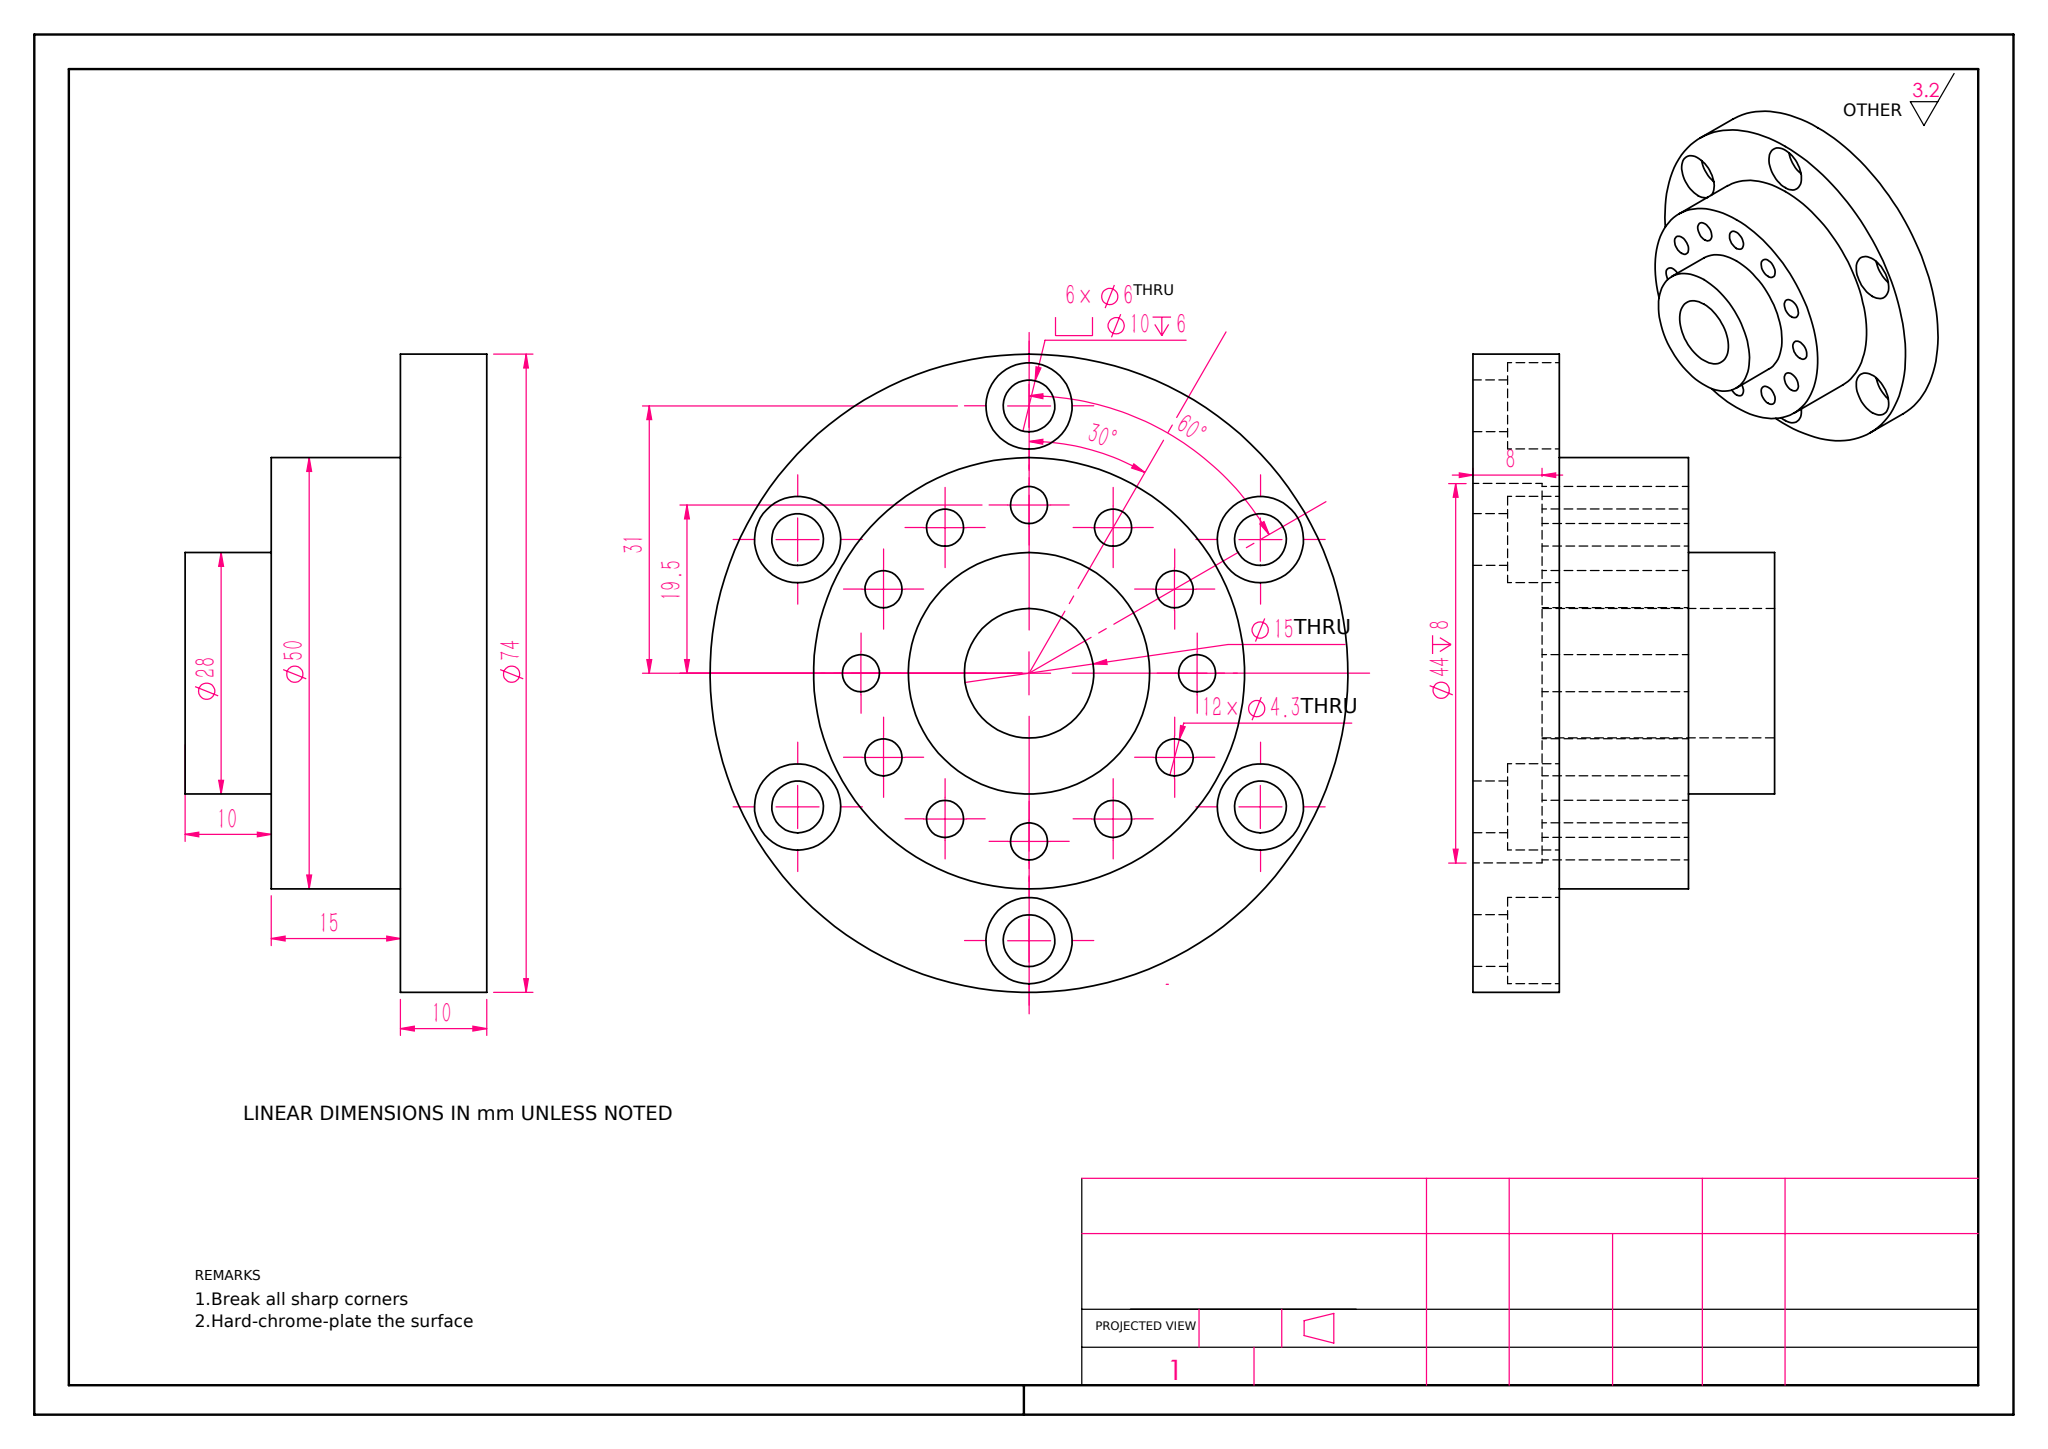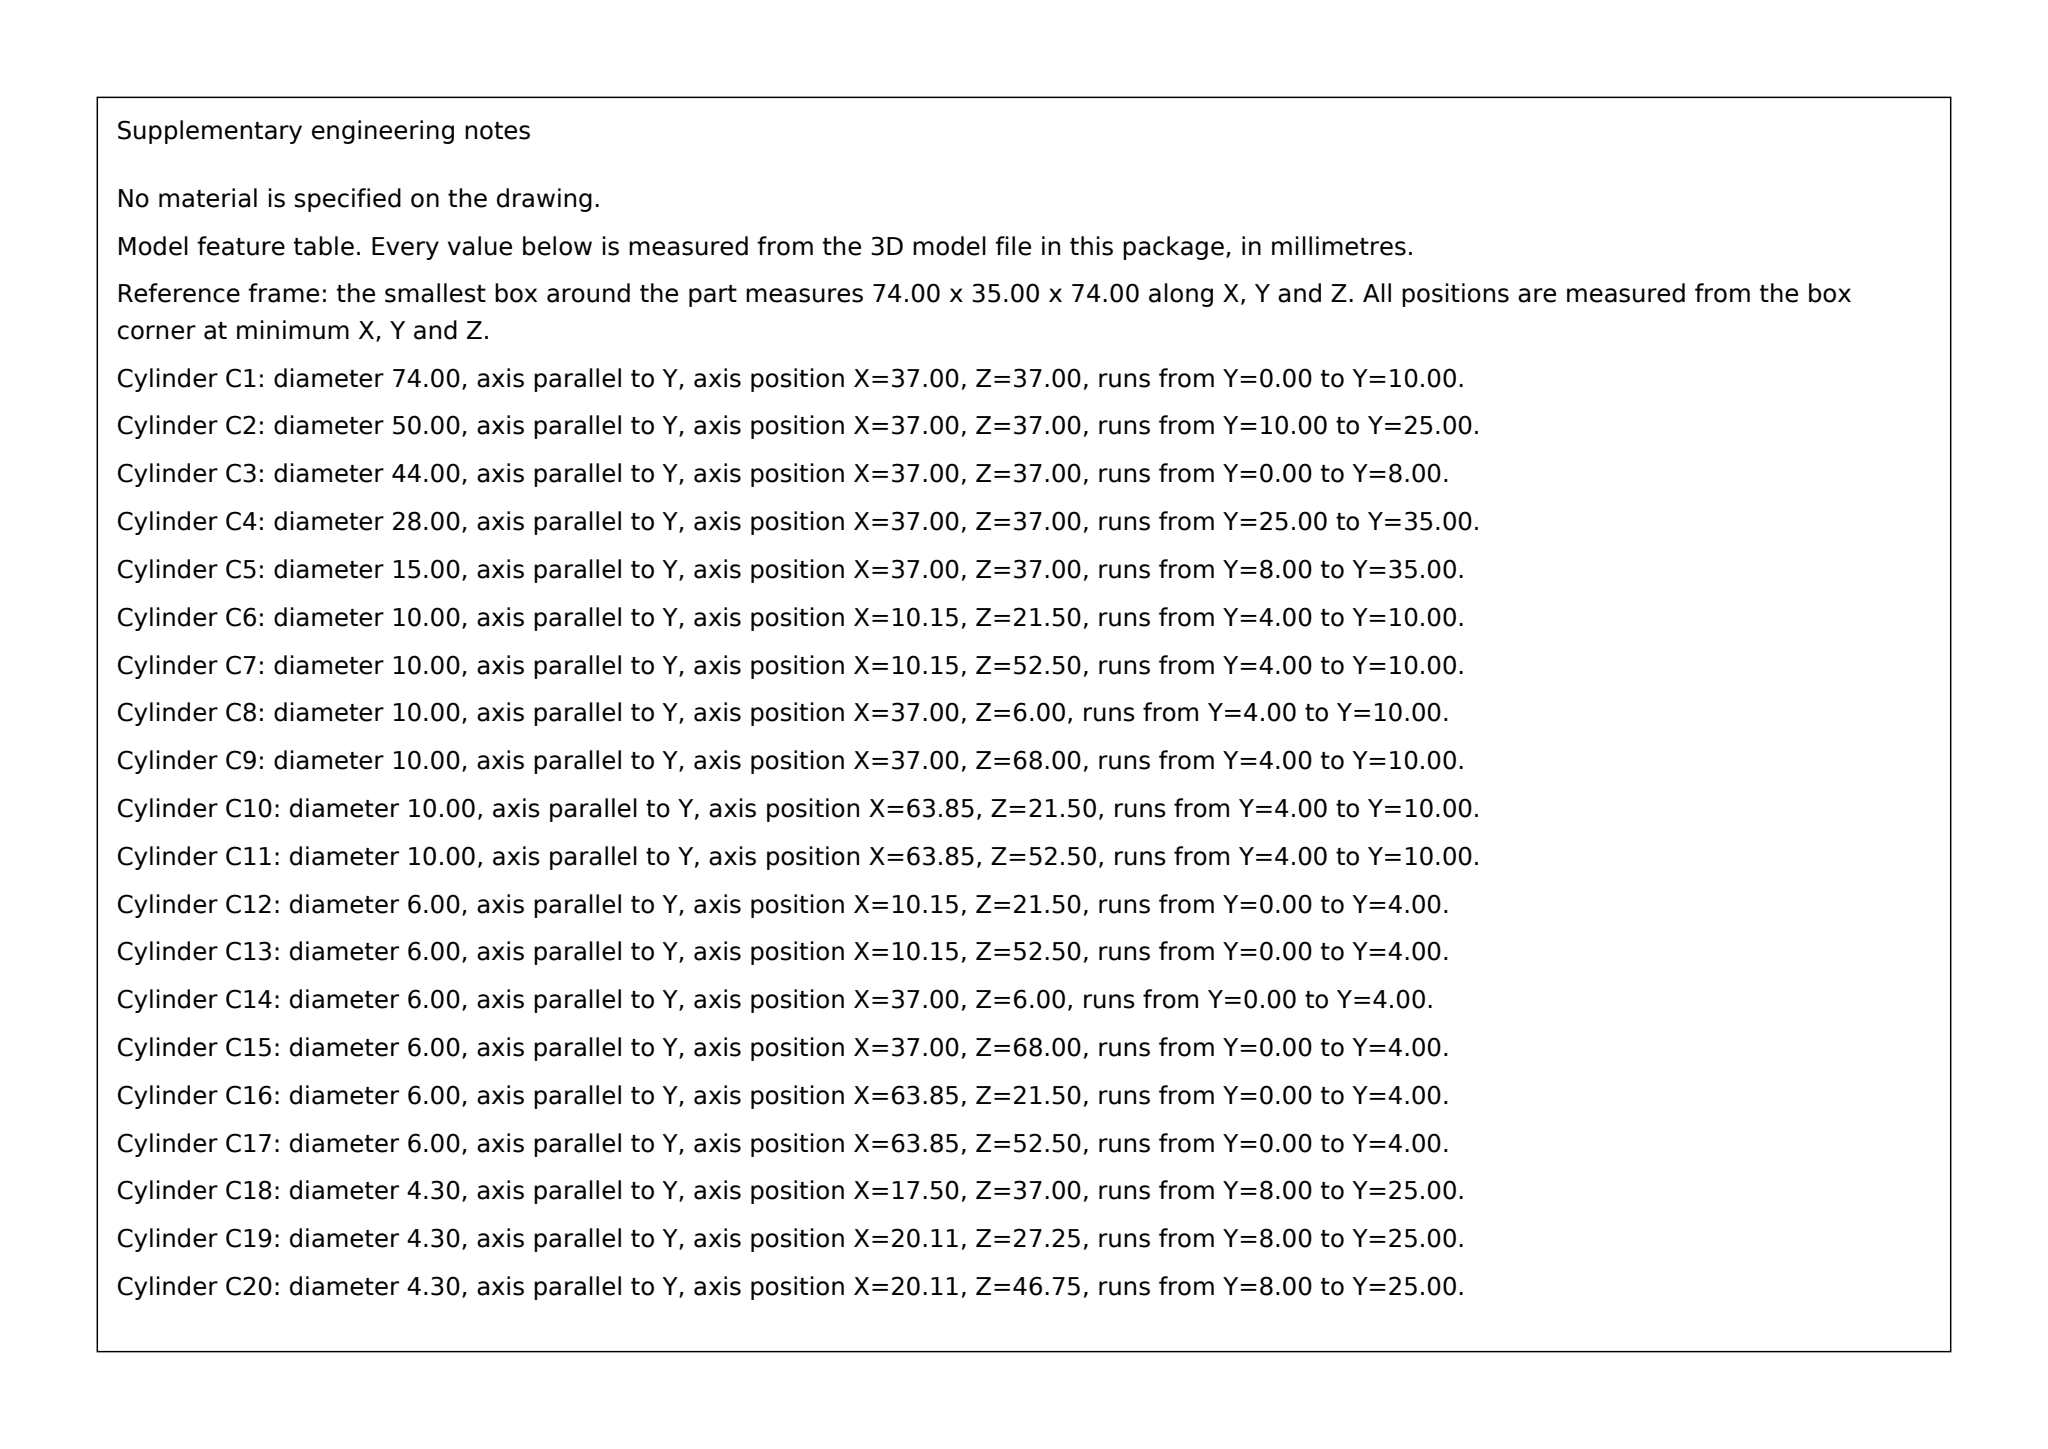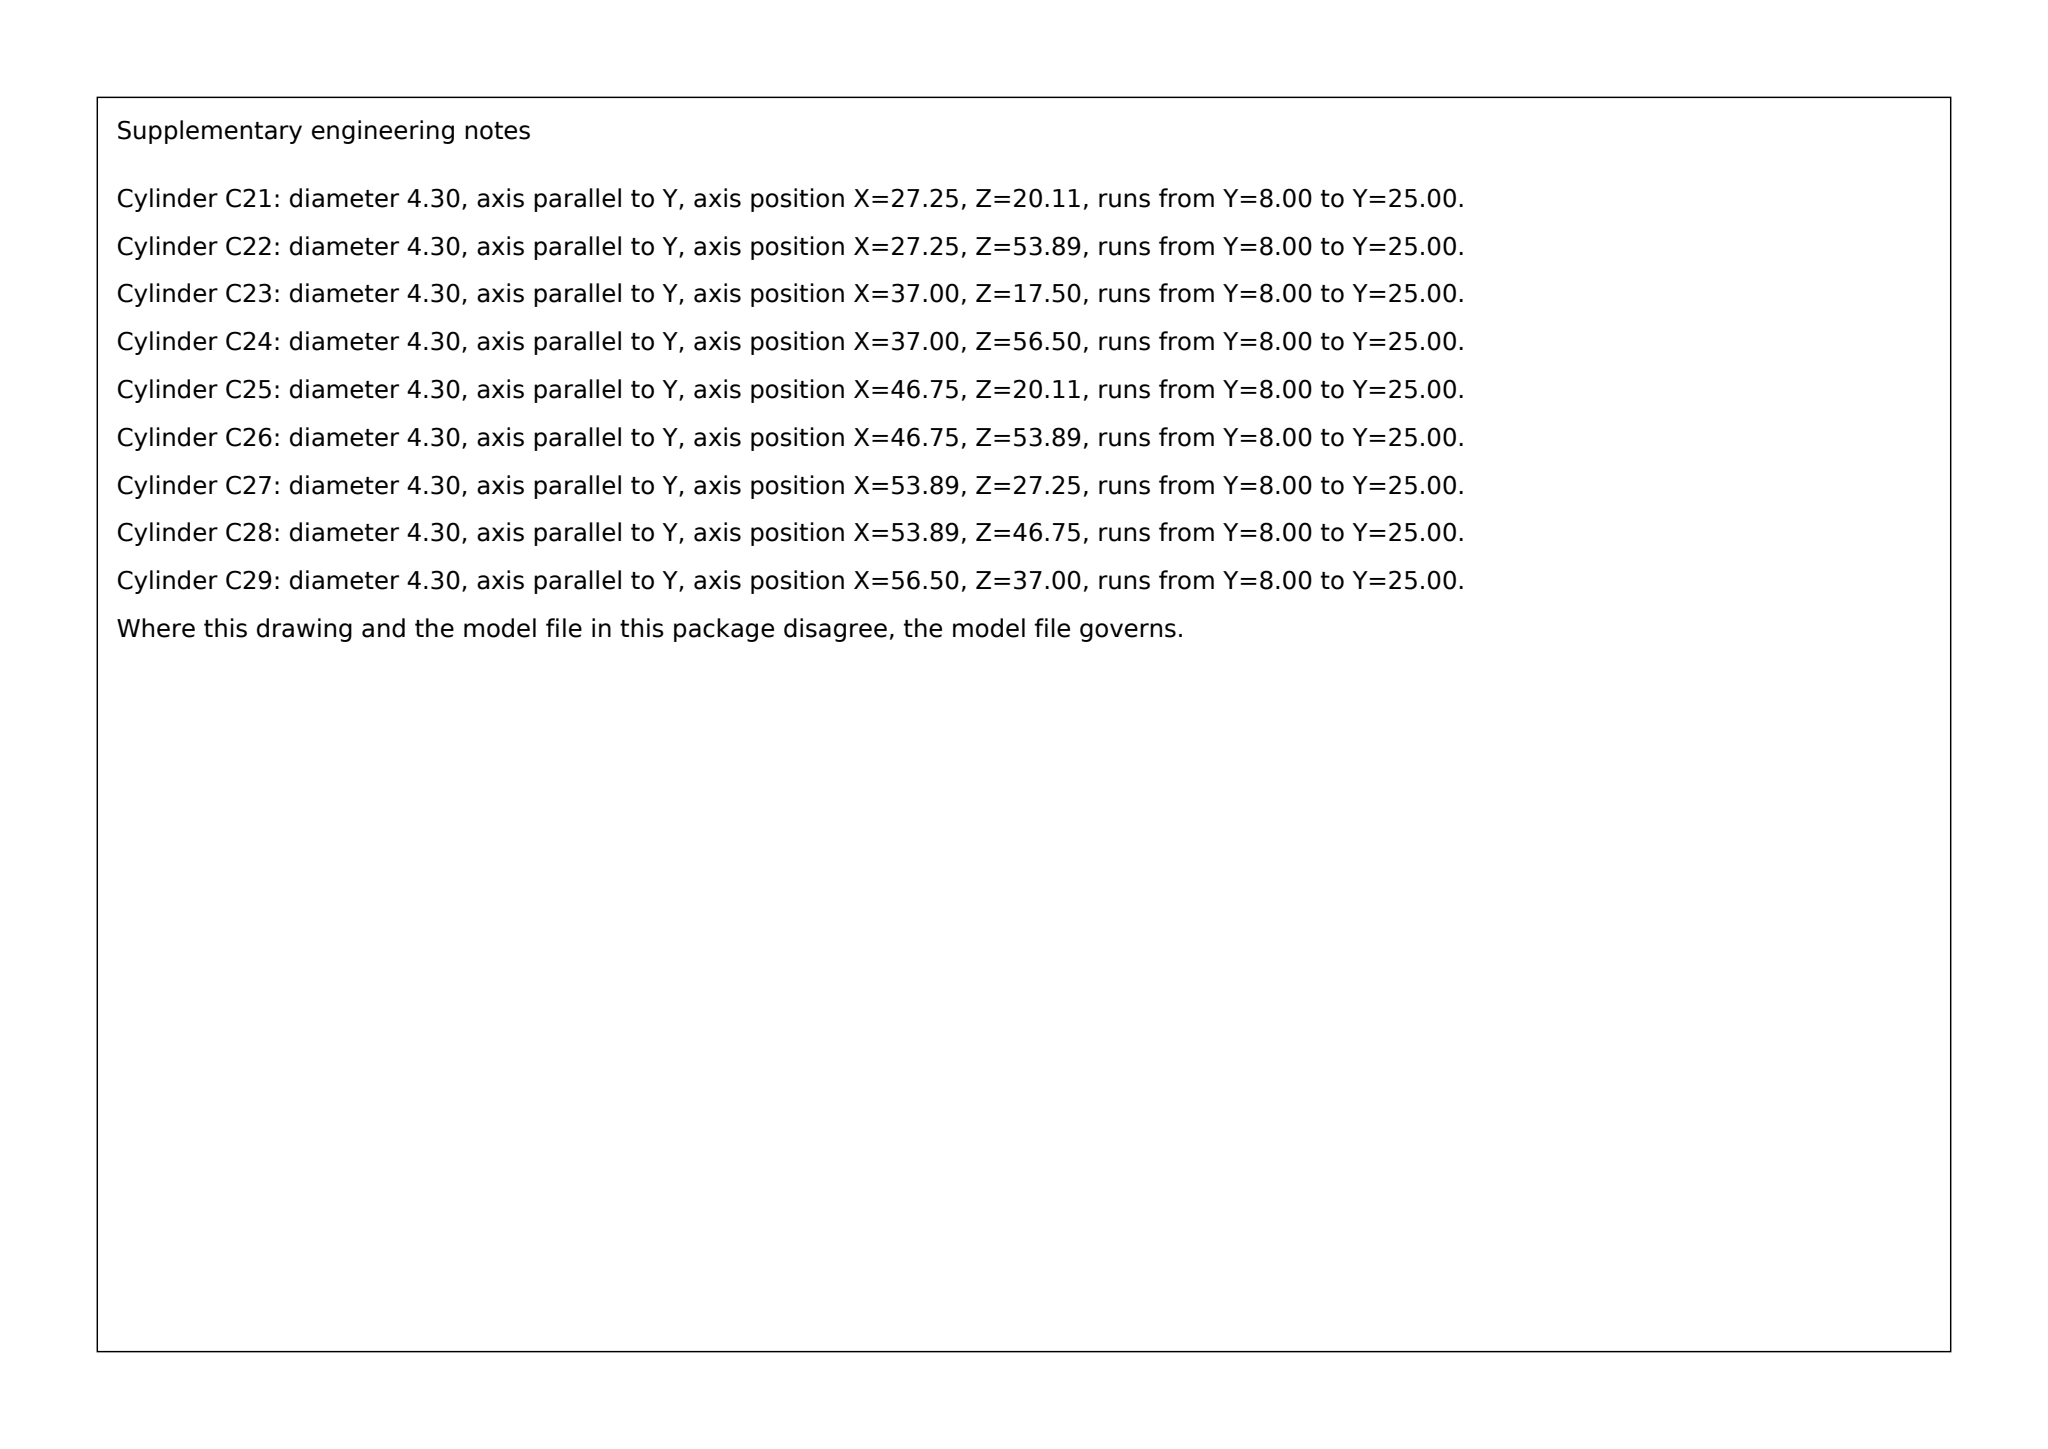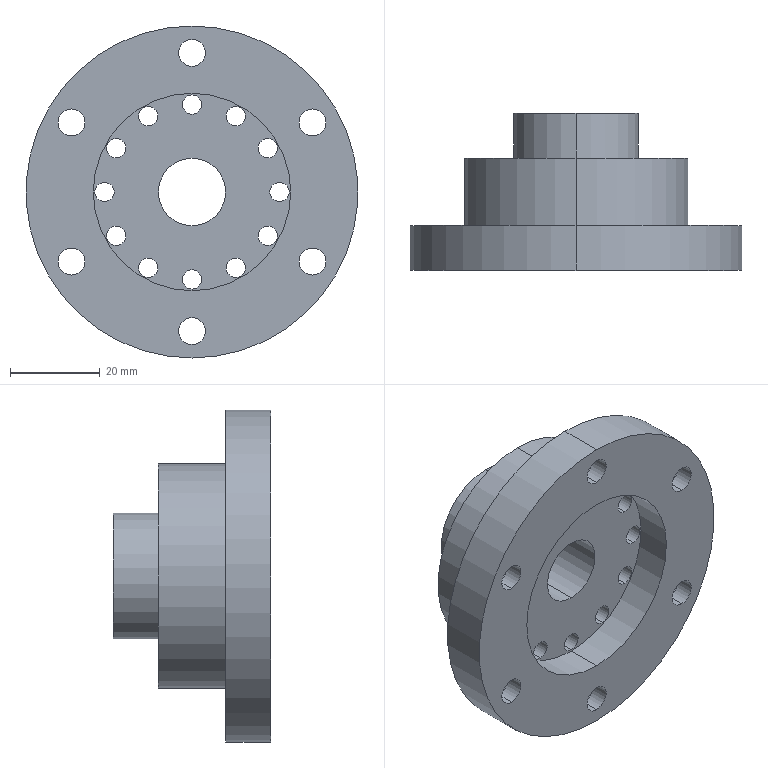Part | SolidWorks | mm | 1 solid | 69 faces | box 74 x 35 x 74 mm | volume 55214 mm3 | cylinder 58 | plane 11 | commonest cylinder face diameters 4.3 x24 10 x12 6 x12 44 x2 50 x2 74 x2 28 x2 15 x2
build123d program:
from build123d import *

# Parameters (mm, degrees)
SKETCH2_R          = 3
CUT_EXTRUDE1_DEPTH = 58.991
SKETCH3_R          = 5
CUT_EXTRUDE2_DEPTH = 6
SKETCH4_R          = 2.15
CUT_EXTRUDE3_DEPTH = 58.991
SKETCH5_R          = 22
CUT_EXTRUDE4_DEPTH = 8


with BuildPart() as part:
    # Sketch1 → Revolve1 (revolve)
    with BuildSketch(Plane.XY, mode=Mode.PRIVATE) as revolve1_sk:
        Polygon((-7.5, 52.197), (-14, 52.197), (-14, 42.197), (-25, 42.197), (-25, 27.197), (-37, 27.197), (-37, 17.197), (-7.5, 17.197), align=None)
    revolve(revolve1_sk.sketch.rotate(Axis((0, 52.197, 0), (0, 1, 0)), 270), axis=Axis((0, 52.197, 0), (0, 1, 0)))

    # Sketch2 → Cut-Extrude1 (cut, through all)
    with BuildSketch(Plane(origin=(0, 27.197, 0), x_dir=(1, 0, 0), z_dir=(0, 1, 0))):
        with Locations(Location((0, 31, 0), (0, 0, 270))):
            Circle(SKETCH2_R)
        with Locations(Location((26.847, 15.5, 0), (0, 0, 270))):
            Circle(SKETCH2_R)
        with Locations(Location((26.847, -15.5, 0), (0, 0, 270))):
            Circle(SKETCH2_R)
        with Locations(Location((0, -31, 0), (0, 0, 270))):
            Circle(SKETCH2_R)
        with Locations(Location((-26.847, -15.5, 0), (0, 0, 270))):
            Circle(SKETCH2_R)
        with Locations(Location((-26.847, 15.5, 0), (0, 0, 270))):
            Circle(SKETCH2_R)
    extrude(amount=-CUT_EXTRUDE1_DEPTH, mode=Mode.SUBTRACT)

    # Sketch3 → Cut-Extrude2 (cut)
    with BuildSketch(Plane(origin=(0, 27.197, 0), x_dir=(1, 0, 0), z_dir=(0, 1, 0))):
        with Locations(Location((0, 31, 0), (0, 0, 270))):
            Circle(SKETCH3_R)
        with Locations(Location((26.847, 15.5, 0), (0, 0, 270))):
            Circle(SKETCH3_R)
        with Locations(Location((26.847, -15.5, 0), (0, 0, 270))):
            Circle(SKETCH3_R)
        with Locations(Location((0, -31, 0), (0, 0, 270))):
            Circle(SKETCH3_R)
        with Locations(Location((-26.847, -15.5, 0), (0, 0, 270))):
            Circle(SKETCH3_R)
        with Locations(Location((-26.847, 15.5, 0), (0, 0, 270))):
            Circle(SKETCH3_R)
    extrude(amount=-CUT_EXTRUDE2_DEPTH, mode=Mode.SUBTRACT)

    # Sketch4 → Cut-Extrude3 (cut, through all)
    with BuildSketch(Plane(origin=(0, 42.197, 0), x_dir=(1, 0, 0), z_dir=(0, 1, 0))):
        with Locations(Location((0, 19.5, 0), (0, 0, 270))):
            Circle(SKETCH4_R)
        with Locations(Location((9.75, 16.887, 0), (0, 0, 270))):
            Circle(SKETCH4_R)
        with Locations(Location((16.887, 9.75, 0), (0, 0, 270))):
            Circle(SKETCH4_R)
        with Locations(Location((19.5, 0, 0), (0, 0, 270))):
            Circle(SKETCH4_R)
        with Locations(Location((16.887, -9.75, 0), (0, 0, 270))):
            Circle(SKETCH4_R)
        with Locations(Location((9.75, -16.887, 0), (0, 0, 270))):
            Circle(SKETCH4_R)
        with Locations(Location((0, -19.5, 0), (0, 0, 270))):
            Circle(SKETCH4_R)
        with Locations(Location((-9.75, -16.887, 0), (0, 0, 270))):
            Circle(SKETCH4_R)
        with Locations(Location((-16.887, -9.75, 0), (0, 0, 270))):
            Circle(SKETCH4_R)
        with Locations(Location((-19.5, 0, 0), (0, 0, 270))):
            Circle(SKETCH4_R)
        with Locations(Location((-16.887, 9.75, 0), (0, 0, 270))):
            Circle(SKETCH4_R)
        with Locations(Location((-9.75, 16.887, 0), (0, 0, 270))):
            Circle(SKETCH4_R)
    extrude(amount=-CUT_EXTRUDE3_DEPTH, mode=Mode.SUBTRACT)

    # Sketch5 → Cut-Extrude4 (cut)
    with BuildSketch(Plane.XZ.offset(-17.197)):
        with Locations(Location((0, 0, 0), (0, 0, 270))):
            Circle(SKETCH5_R)
    extrude(amount=-CUT_EXTRUDE4_DEPTH, mode=Mode.SUBTRACT)


solid = part.part